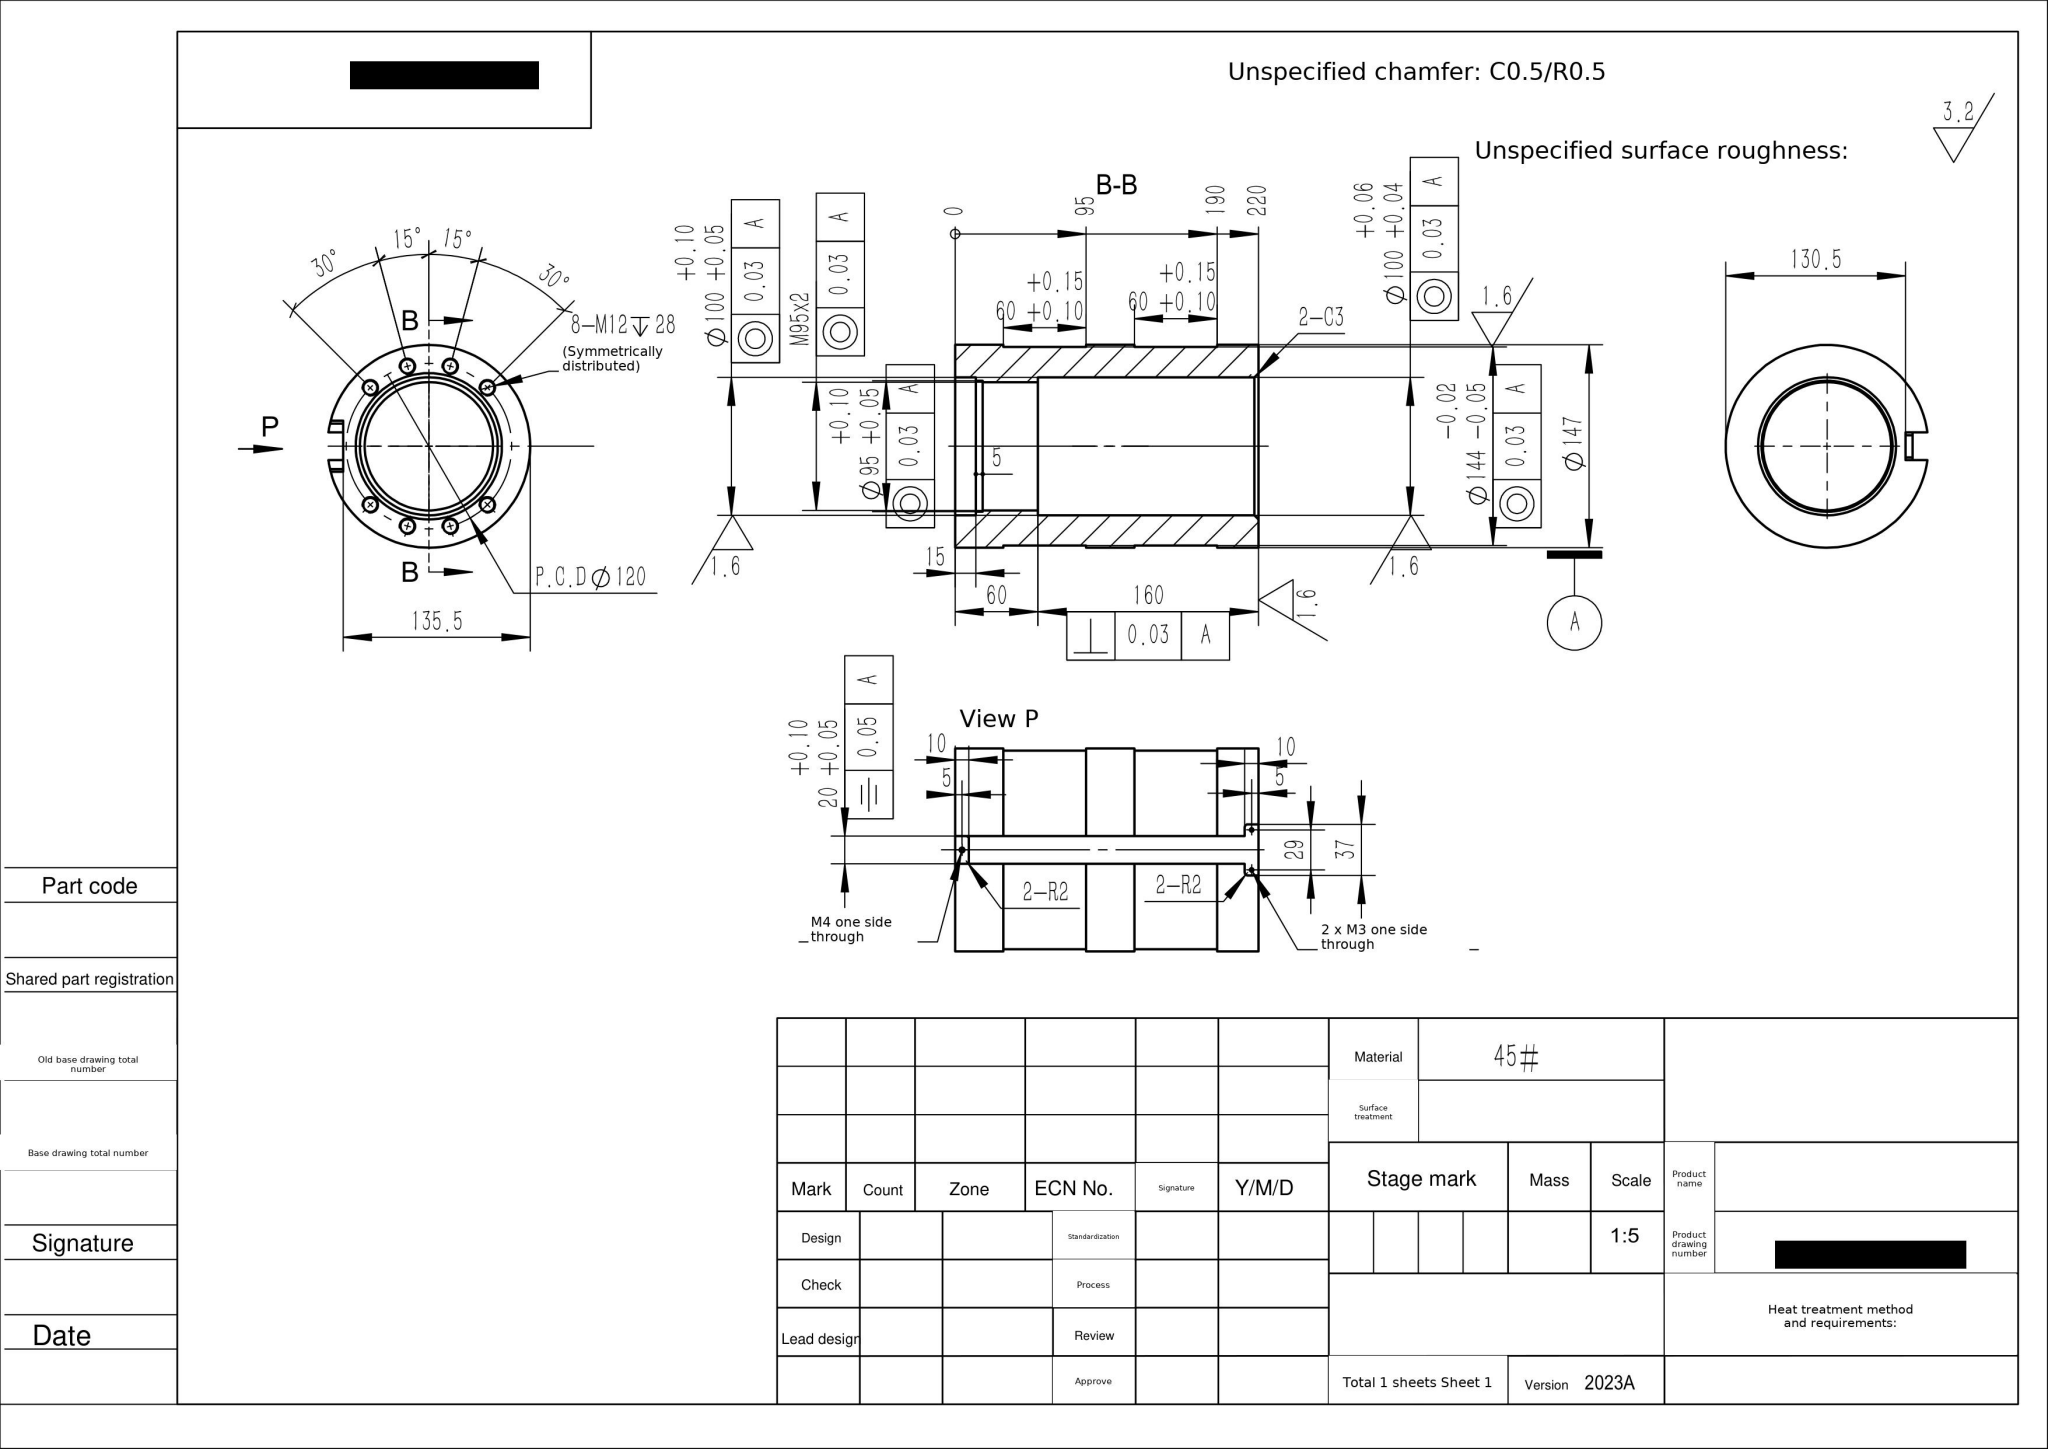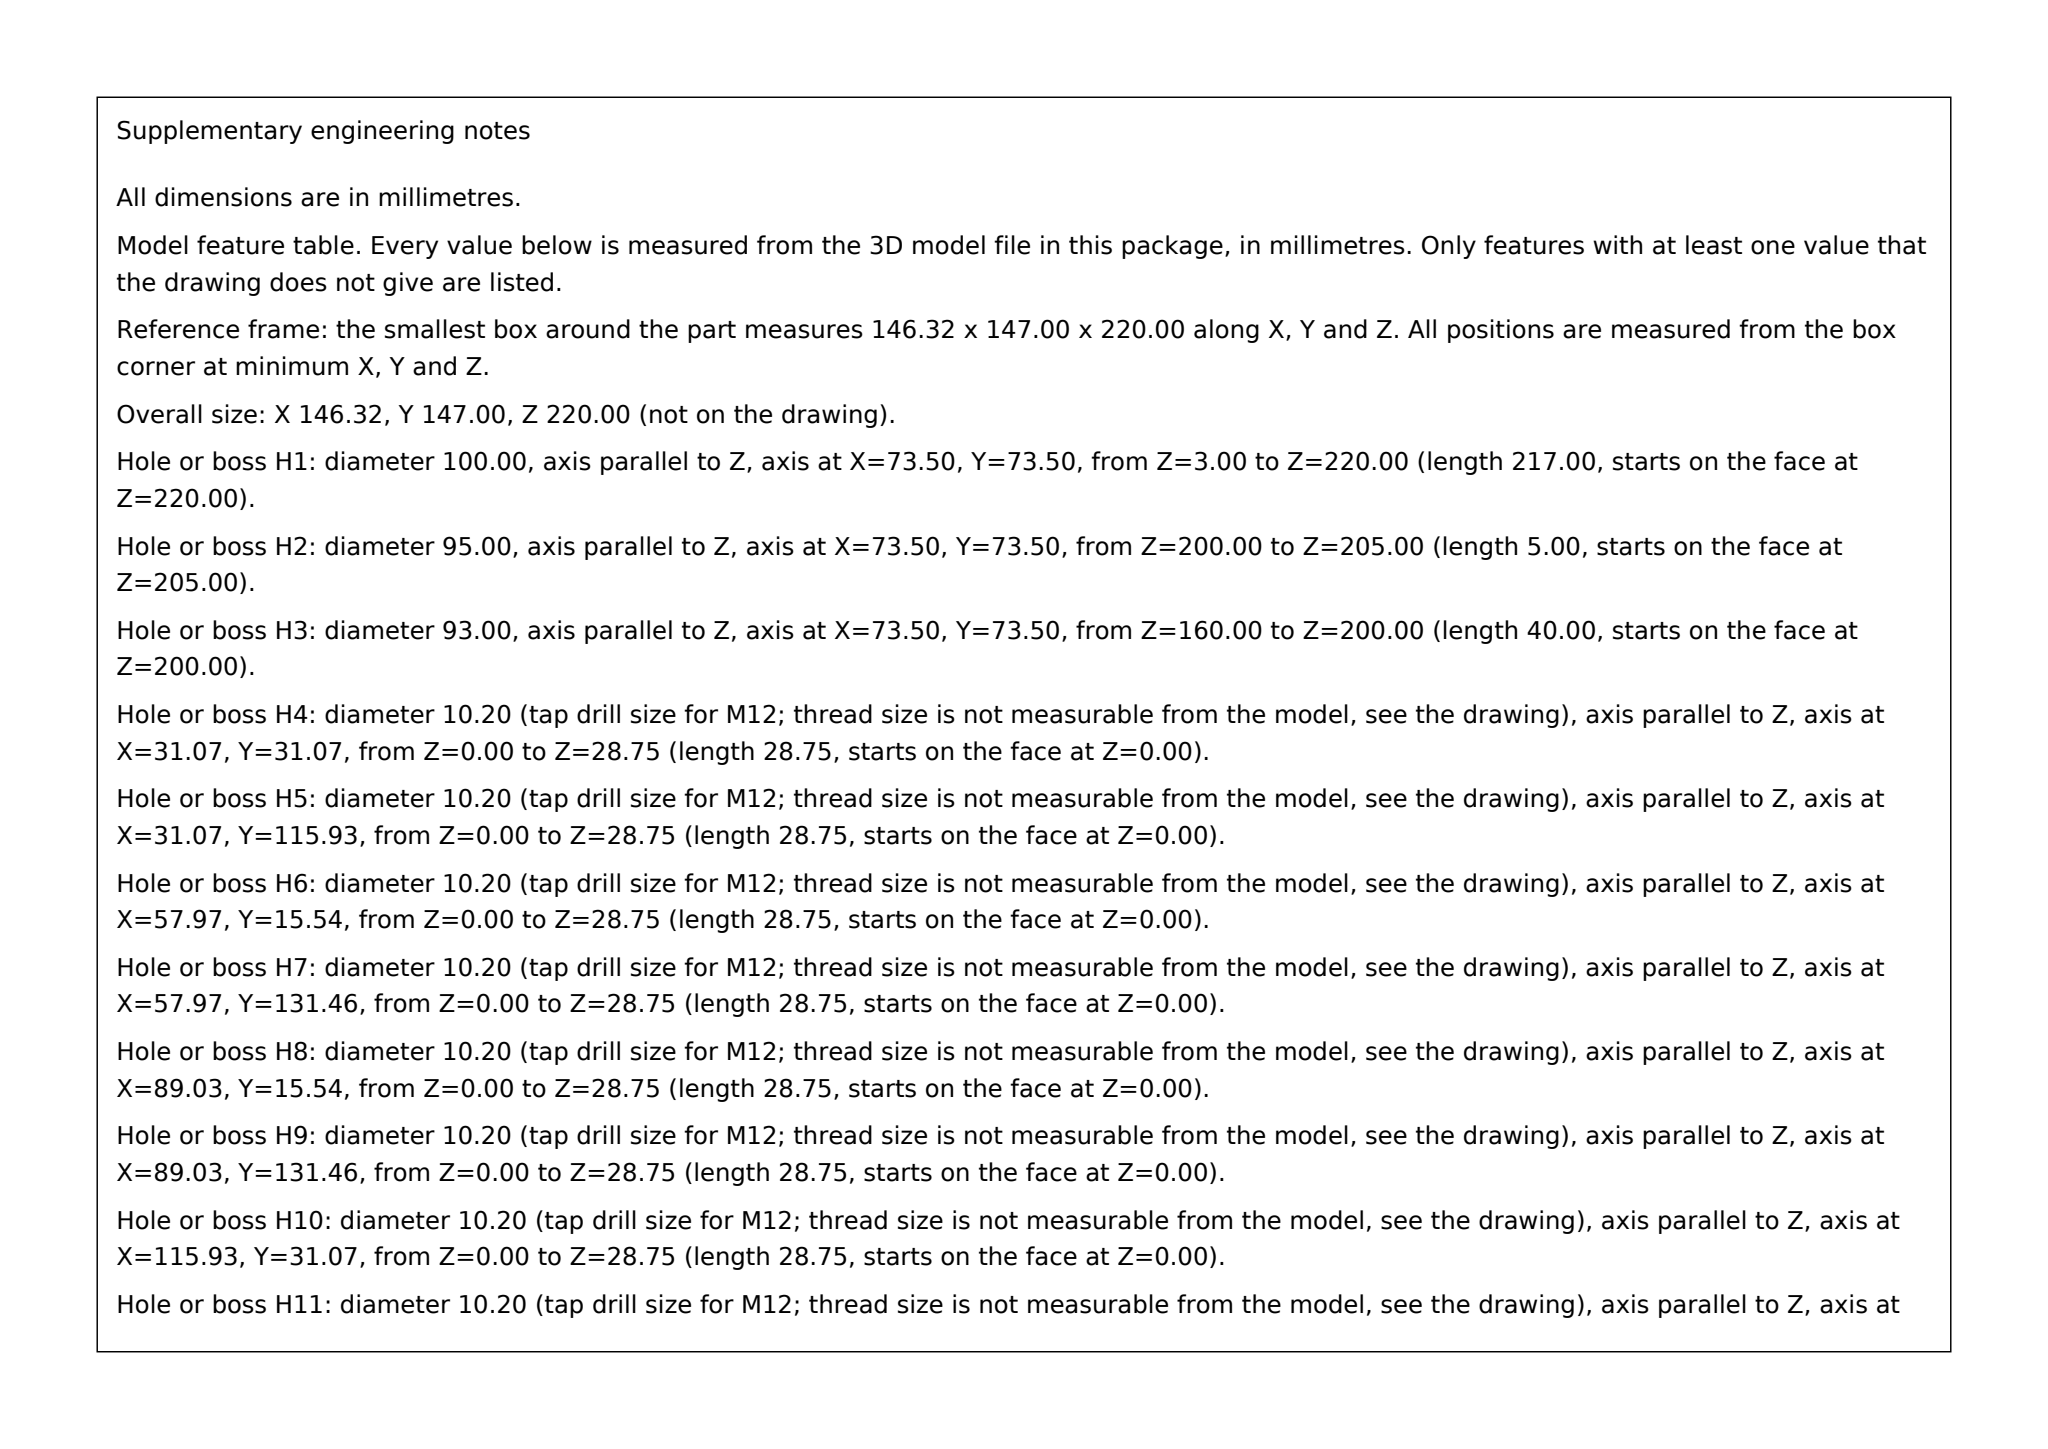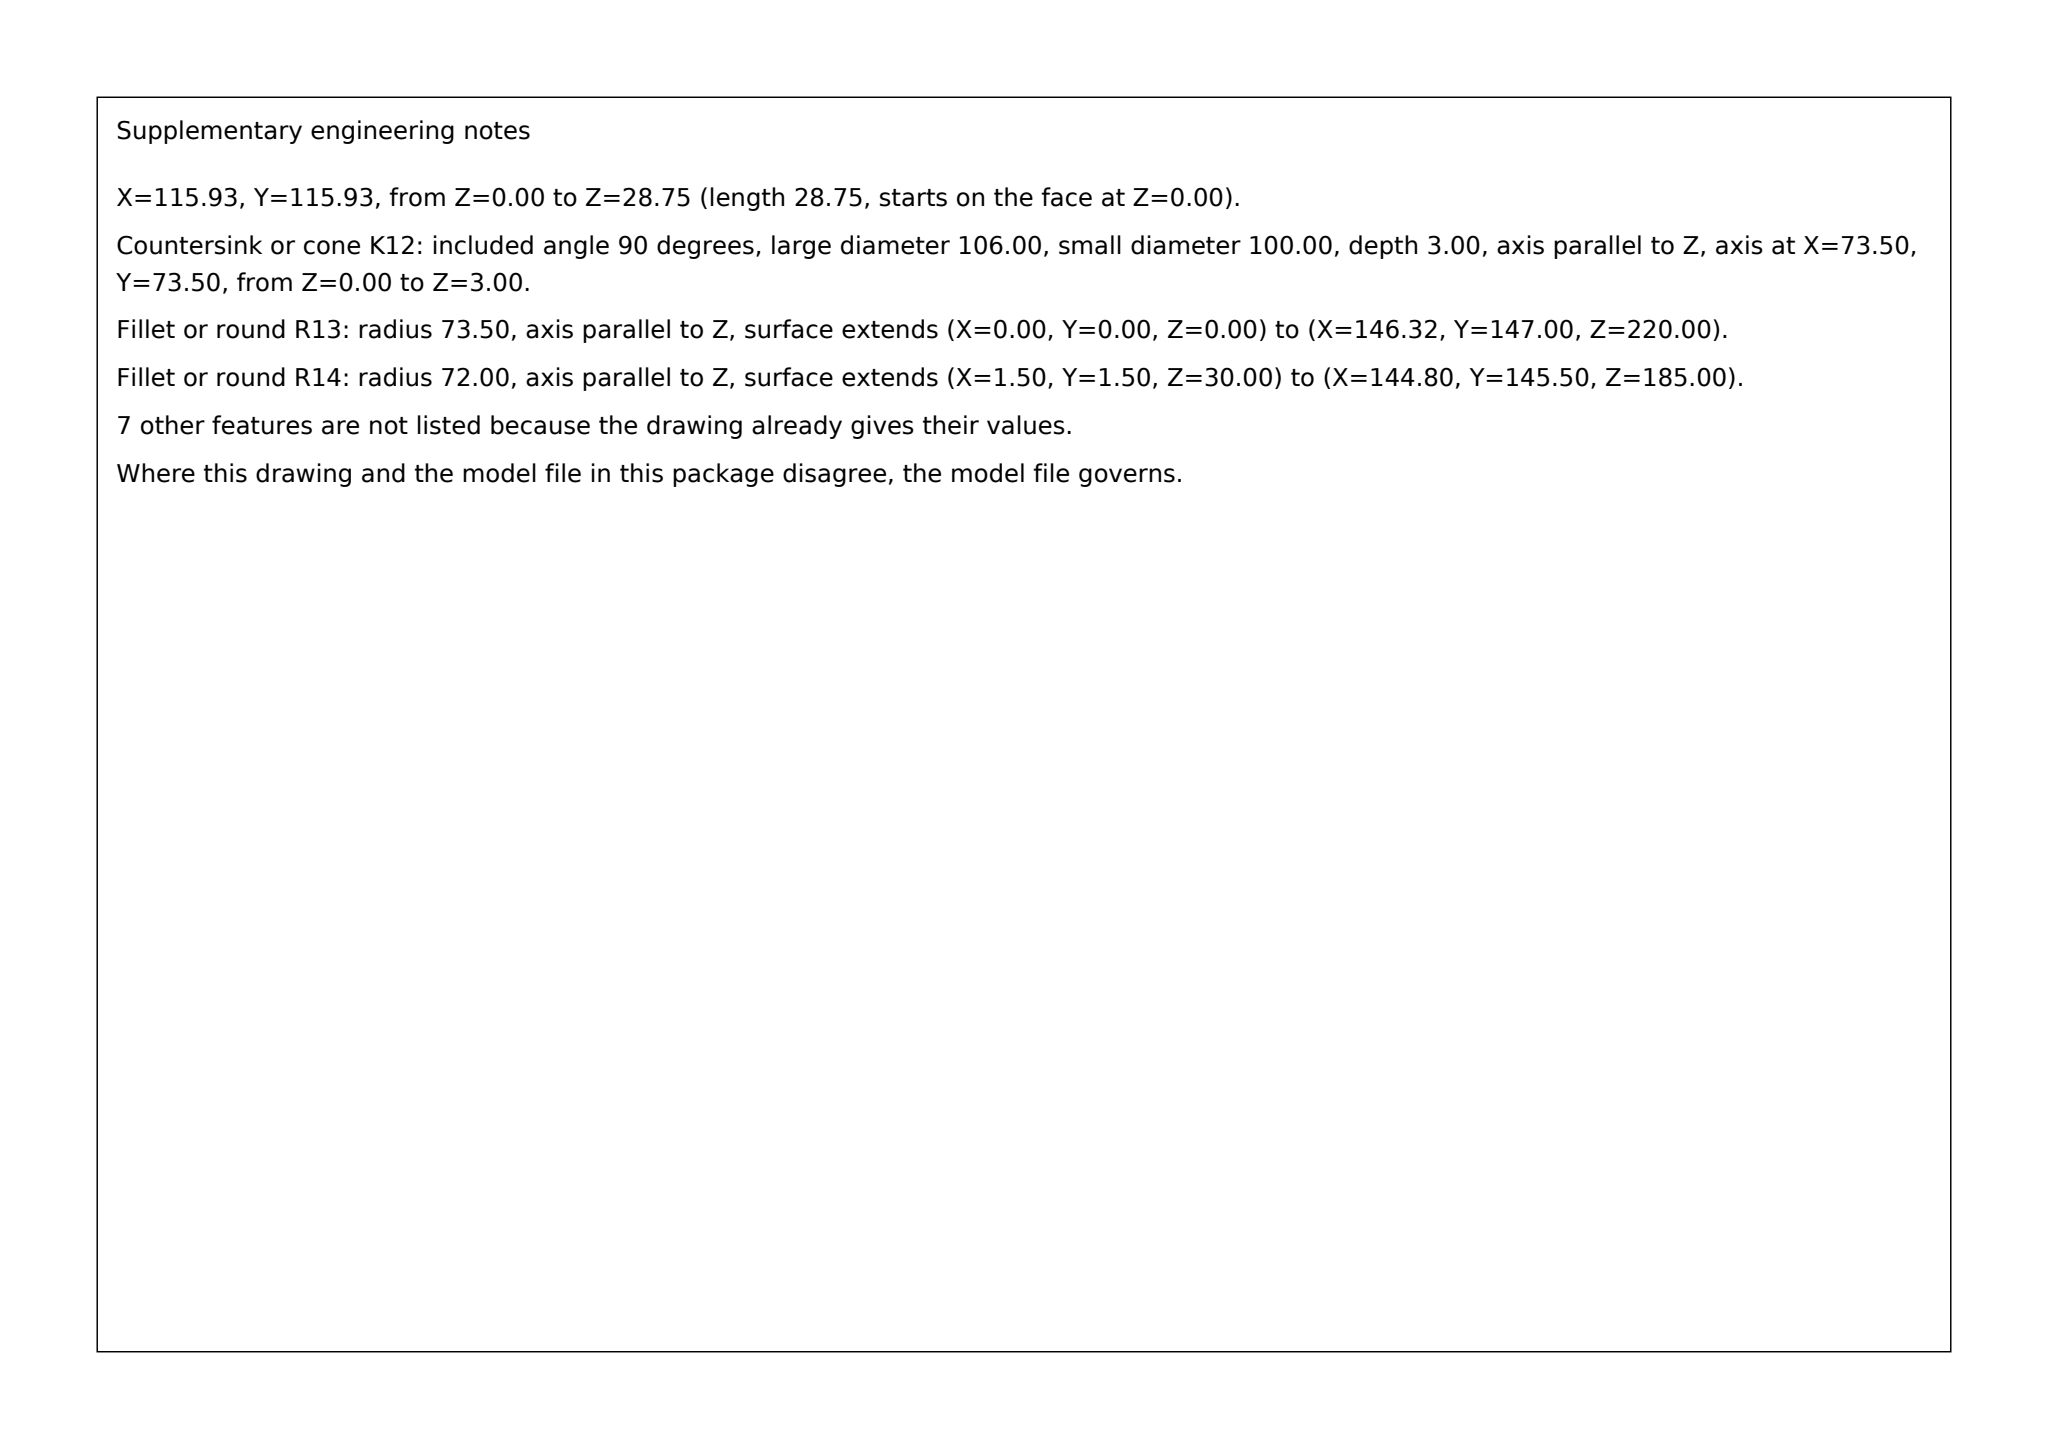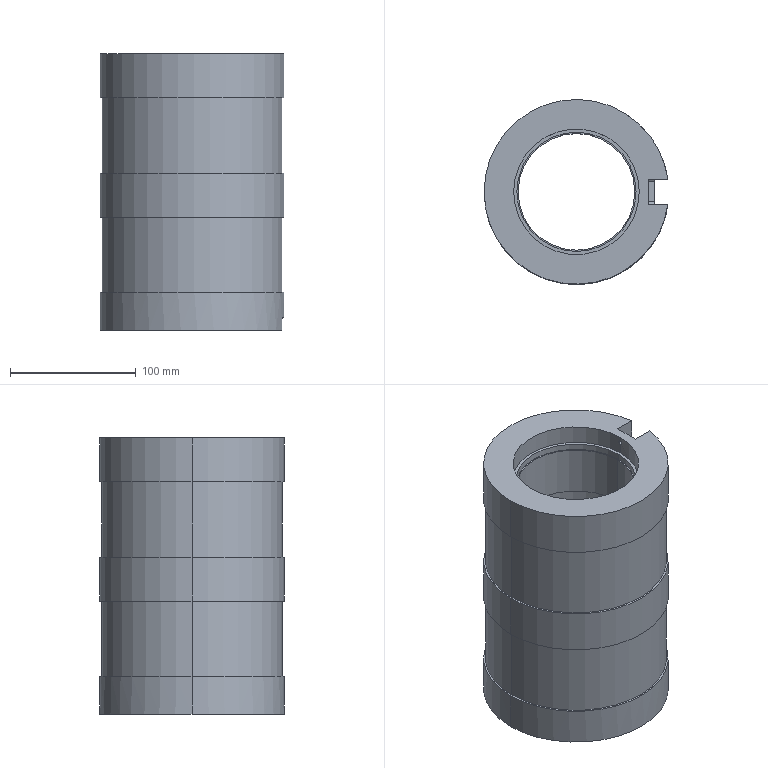Part | SolidWorks | mm | material 45# | 1 solid | 80 faces | box 146.32 x 147 x 220 mm | volume 1900108 mm3 | cylinder 44 | cone 18 | plane 18 | commonest cylinder face diameters 10.2 x16 147 x6 100 x4 2.5 x4 144 x4 4 x4 95 x2 3.3 x2
build123d program:
from build123d import *

# Parameters (mm, degrees)
SKETCH1_R                   = 73.5
SKETCH1_R_2                 = 46.5
BOSS_EXTRUDE1_DEPTH         = 230
SKETCH2_W                   = 20
SKETCH2_H                   = 20
CUT_EXTRUDE1_DEPTH          = 253.398
M12_TAPPED_HOLE1_AT_2_COUNT = 2
M12_TAPPED_HOLE1_AT_2_PITCH = 31.058
M12_TAPPED_HOLE1_AT_3_COUNT = 2
M12_TAPPED_HOLE1_AT_3_PITCH = 60
M12_TAPPED_HOLE1_AT_4_COUNT = 2
M12_TAPPED_HOLE1_AT_4_PITCH = 31.058
SKETCH8_W                   = 10
SKETCH8_H                   = 20
CUT_EXTRUDE4_DEPTH          = 5
CUT_EXTRUDE6_START          = -40
SKETCH11_2_R                = 90
SKETCH11_2_R_2              = 72
CUT_EXTRUDE6_DEPTH          = 60
CUT_EXTRUDE7_START          = -135
SKETCH11_2_2_R              = 90
SKETCH11_2_2_R_2            = 72
CUT_EXTRUDE7_DEPTH          = 60
FILLET1_R                   = 2
M4_TAPPED_HOLE1_D           = 3.3
M4_TAPPED_HOLE1_DEPTH       = 11.5
M4_TAPPED_HOLE1_TIP         = 0.9914
SKETCH15_W                  = 25
SKETCH15_H                  = 37
CUT_EXTRUDE8_DEPTH          = 277.88
FILLET2_R                   = 2
M3_TAPPED_HOLE1_D           = 2.5
M3_TAPPED_HOLE1_DEPTH       = 22.5
M3_TAPPED_HOLE1_TIP         = 0.7511
SKETCH19_R                  = 50
CUT_EXTRUDE9_DEPTH          = 170
CUT_EXTRUDE10_START         = -15
SKETCH20_R                  = 50
CUT_EXTRUDE10_DEPTH         = 15
SKETCH21_R                  = 176.703
CUT_EXTRUDE11_DEPTH         = 10
CHAMFER1_SIZE               = 1
CHAMFER2_SIZE               = 3
SKETCH22_R                  = 47.5
CUT_EXTRUDE12_DEPTH         = 5


with BuildPart() as part:
    # Sketch1 → Boss-Extrude1 (new body)
    with BuildSketch(Plane.XY):
        Circle(SKETCH1_R)
        Circle(SKETCH1_R_2, mode=Mode.SUBTRACT)
    extrude(amount=BOSS_EXTRUDE1_DEPTH)

    # Sketch2 → Cut-Extrude1 (cut, through all)
    with BuildSketch(Plane(origin=(0, 0, 0), x_dir=(-1, 0, 0), z_dir=(0, 0, -1))):
        with Locations((-72, 0)):
            Rectangle(SKETCH2_W, SKETCH2_H)
    extrude(amount=-CUT_EXTRUDE1_DEPTH, mode=Mode.SUBTRACT)

    # Sketch3 → M12 Tapped Hole1 (revolve, cut)
    with BuildSketch(Plane(origin=(-15.529, 57.956, 0), x_dir=(0, 1, 0), z_dir=(1, 0, 0))):
        Polygon((0, 0), (0, 41.814), (5.1, 38.75), (5.1, 0), align=None)
    m12_tapped_hole1 = revolve(axis=Axis((-15.529, 57.956, -6.35), (0, 0, 1)), mode=Mode.SUBTRACT)

    # M12 Tapped Hole1 at 2: M12 Tapped Hole1 ×2
    with Locations(*[Vector(-0.866, -0.5, 0) * (i * M12_TAPPED_HOLE1_AT_2_PITCH) for i in range(1, M12_TAPPED_HOLE1_AT_2_COUNT)]):
        add(m12_tapped_hole1, mode=Mode.SUBTRACT)

    # M12 Tapped Hole1 at 3: M12 Tapped Hole1 ×2
    with Locations(*[Vector(0.9659, -0.2588, 0) * (i * M12_TAPPED_HOLE1_AT_3_PITCH) for i in range(1, M12_TAPPED_HOLE1_AT_3_COUNT)]):
        add(m12_tapped_hole1, mode=Mode.SUBTRACT)

    # M12 Tapped Hole1 at 4: M12 Tapped Hole1 ×2
    with Locations(*[(i * M12_TAPPED_HOLE1_AT_4_PITCH, 0, 0) for i in range(1, M12_TAPPED_HOLE1_AT_4_COUNT)]):
        add(m12_tapped_hole1, mode=Mode.SUBTRACT)

    # Sketch8 → Cut-Extrude4 (cut)
    with BuildSketch(Plane(origin=(62, 0, 0), x_dir=(0, 0, -1), z_dir=(1, 0, 0))):
        with Locations((-225, 0)):
            Rectangle(SKETCH8_W, SKETCH8_H)
    extrude(amount=-CUT_EXTRUDE4_DEPTH, mode=Mode.SUBTRACT)

    # Sketch11_2 → Cut-Extrude6 (cut)
    with BuildSketch(Plane(origin=(0, 0, 0), x_dir=(-1, 0, 0), z_dir=(0, 0, -1)).offset(CUT_EXTRUDE6_START)):
        Circle(SKETCH11_2_R)
        Circle(SKETCH11_2_R_2, mode=Mode.SUBTRACT)
    extrude(amount=-CUT_EXTRUDE6_DEPTH, mode=Mode.SUBTRACT)

    # Sketch11_2 2 → Cut-Extrude7 (cut)
    with BuildSketch(Plane(origin=(0, 0, 0), x_dir=(-1, 0, 0), z_dir=(0, 0, -1)).offset(CUT_EXTRUDE7_START)):
        Circle(SKETCH11_2_2_R)
        Circle(SKETCH11_2_2_R_2, mode=Mode.SUBTRACT)
    extrude(amount=-CUT_EXTRUDE7_DEPTH, mode=Mode.SUBTRACT)

    # Fillet1
    fillet1_edges = [part.edges().sort_by_distance(p)[0] for p in [
        (59.5, 10, 220),
        (59.5, -10, 220),
    ]]
    fillet(fillet1_edges, radius=FILLET1_R)

    # M4 Tapped Hole1
    with Locations(Plane(origin=(57, 0, 0), x_dir=(0, 0, -1), z_dir=(1, 0, 0))):
        with Locations((-225, 0)):
            Hole(M4_TAPPED_HOLE1_D / 2, depth=M4_TAPPED_HOLE1_DEPTH)
            with Locations((0, 0, -(M4_TAPPED_HOLE1_DEPTH + M4_TAPPED_HOLE1_TIP / 2))):  # 118° drill point
                Cone(0, M4_TAPPED_HOLE1_D / 2, M4_TAPPED_HOLE1_TIP, mode=Mode.SUBTRACT)

    # Sketch15 → Cut-Extrude8 (cut, through all)
    with BuildSketch(Plane(origin=(62, 0, 0), x_dir=(0, 0, -1), z_dir=(1, 0, 0))):
        with Locations((-7.5, 0)):
            Rectangle(SKETCH15_W, SKETCH15_H)
    extrude(amount=CUT_EXTRUDE8_DEPTH, mode=Mode.SUBTRACT)

    # Fillet2
    fillet2_edges = [part.edges().sort_by_distance(p)[0] for p in [
        (66.567, -18.5, 20),
        (66.567, 18.5, 20),
    ]]
    fillet(fillet2_edges, radius=FILLET2_R)

    # M3 Tapped Hole1
    with Locations(Plane(origin=(62, 0, 0), x_dir=(0, 0, -1), z_dir=(1, 0, 0))):
        with Locations((-15, 14.5), (-15, -14.5)):
            Hole(M3_TAPPED_HOLE1_D / 2, depth=M3_TAPPED_HOLE1_DEPTH)
            with Locations((0, 0, -(M3_TAPPED_HOLE1_DEPTH + M3_TAPPED_HOLE1_TIP / 2))):  # 118° drill point
                Cone(0, M3_TAPPED_HOLE1_D / 2, M3_TAPPED_HOLE1_TIP, mode=Mode.SUBTRACT)

    # Sketch19 → Cut-Extrude9 (cut)
    with BuildSketch(Plane(origin=(0, 0, 0), x_dir=(-1, 0, 0), z_dir=(0, 0, -1))):
        Circle(SKETCH19_R)
    extrude(amount=-CUT_EXTRUDE9_DEPTH, mode=Mode.SUBTRACT)

    # Sketch20 → Cut-Extrude10 (cut)
    with BuildSketch(Plane.XY.offset(230).offset(CUT_EXTRUDE10_START)):
        with Locations(Location((0, 0, 0), (0, 0, 180))):
            Circle(SKETCH20_R)
    extrude(amount=CUT_EXTRUDE10_DEPTH, mode=Mode.SUBTRACT)

    # Mirror1: M12 Tapped Hole1 across plane
    add(m12_tapped_hole1.mirror(Plane.ZX), mode=Mode.SUBTRACT)

    # Mirror1 copy 1 sketch → Mirror1 copy 1 (revolve, cut)
    with BuildSketch(Plane(origin=(-42.426, -42.426, 0), x_dir=(0, -1, 0), z_dir=(1, 0, 0))):
        Polygon((0, 0), (0, -41.814), (5.1, -38.75), (5.1, 0), align=None)
    revolve(axis=Axis((-42.426, -42.426, -6.35), (0, 0, -1)), mode=Mode.SUBTRACT)

    # Mirror1 copy 2 sketch → Mirror1 copy 2 (revolve, cut)
    with BuildSketch(Plane(origin=(42.426, -42.426, 0), x_dir=(0, -1, 0), z_dir=(1, 0, 0))):
        Polygon((0, 0), (0, -41.814), (5.1, -38.75), (5.1, 0), align=None)
    revolve(axis=Axis((42.426, -42.426, -6.35), (0, 0, -1)), mode=Mode.SUBTRACT)

    # Mirror1 copy 3 sketch → Mirror1 copy 3 (revolve, cut)
    with BuildSketch(Plane(origin=(15.529, -57.956, 0), x_dir=(0, -1, 0), z_dir=(1, 0, 0))):
        Polygon((0, 0), (0, -41.814), (5.1, -38.75), (5.1, 0), align=None)
    revolve(axis=Axis((15.529, -57.956, -6.35), (0, 0, -1)), mode=Mode.SUBTRACT)

    # Sketch21 → Cut-Extrude11 (cut)
    with BuildSketch(Plane(origin=(0, 0, 0), x_dir=(-1, 0, 0), z_dir=(0, 0, -1))):
        Circle(SKETCH21_R)
    extrude(amount=-CUT_EXTRUDE11_DEPTH, mode=Mode.SUBTRACT)

    # Chamfer1
    chamfer1_edges = [part.edges().sort_by_distance(p)[0] for p in [
        (-46.5, 0, 215),
    ]]
    chamfer(chamfer1_edges, length=CHAMFER1_SIZE)

    # Chamfer2
    chamfer2_edges = [part.edges().sort_by_distance(p)[0] for p in [
        (50, 0, 10),
    ]]
    chamfer(chamfer2_edges, length=CHAMFER2_SIZE)

    # Sketch22 → Cut-Extrude12 (cut)
    with BuildSketch(Plane.XY.offset(215)):
        Circle(SKETCH22_R)
    extrude(amount=-CUT_EXTRUDE12_DEPTH, mode=Mode.SUBTRACT)


solid = part.part